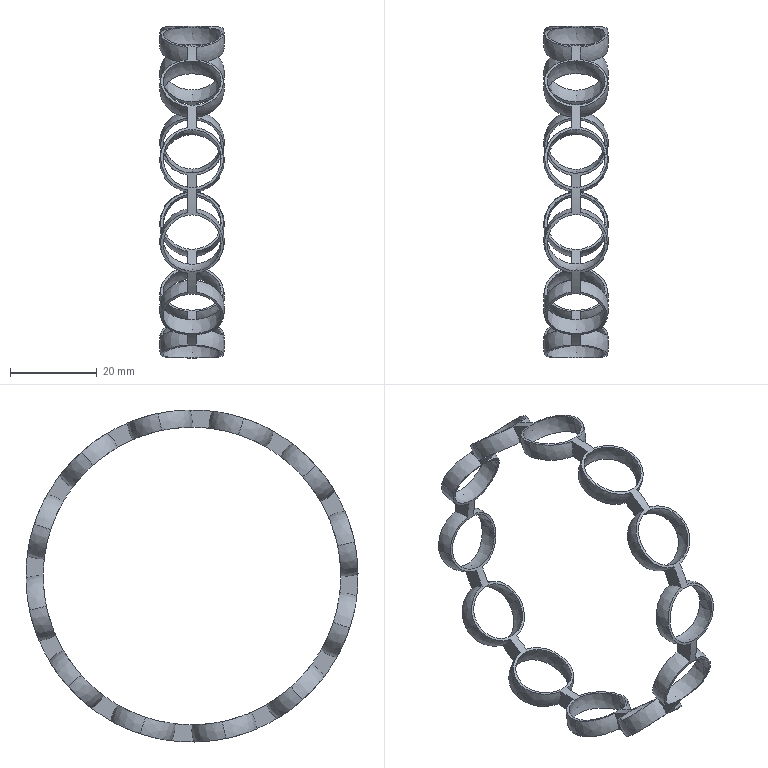Component | SolidWorks | UpperHousingAssembly-1_WormAxisAssembly-1_DeepGrooveBallBearing6309-1_Cage-1 | 1 solid | 100 faces | volume 1601 mm3 | sphere 72 | plane 24 | cylinder 4 | commonest cylinder face diameters 76.5 x2 68.5 x2